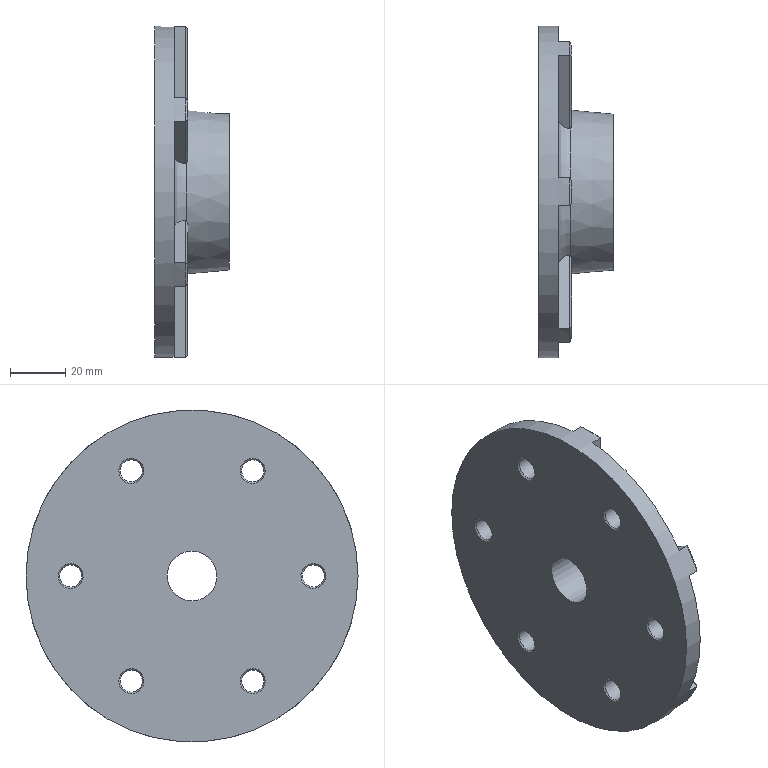Component | NX | FRONT_CASING_COVER | 1 solid | 80 faces | volume 131508 mm3 | plane 38 | cone 25 | cylinder 11 | torus 6 | commonest cylinder face diameters 8 x6 6 x3 120 x1 18 x1